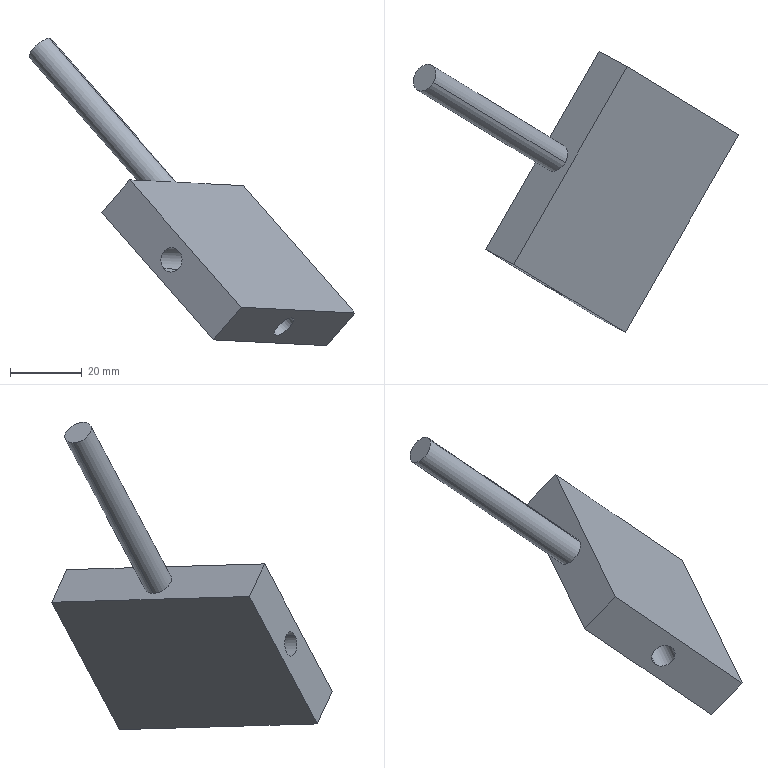Component | SolidWorks | GravitySensorZ0-123-1 | 1 solid | 18 faces | box 90.67 x 78.15 x 85.57 mm | volume 40042 mm3 | cylinder 10 | plane 8 | commonest cylinder face diameters 6.8 x8 8 x2
build123d program:
from build123d import *

# Parameters (mm, degrees)
SKETCH1_W           = 63.5
SKETCH1_H           = 50.8
BOSS_EXTRUDE1_DEPTH = 12.7
M8_TAPPED_HOLE1_D   = 6.8
M8_TAPPED_HOLE2_D   = 6.8
SKETCH6_R           = 4
BOSS_EXTRUDE2_DEPTH = 60


with BuildPart() as part:
    # Sketch1 → Boss-Extrude1 (new body)
    with BuildSketch(Plane.XY):
        Rectangle(SKETCH1_W, SKETCH1_H)
    extrude(amount=BOSS_EXTRUDE1_DEPTH)

    # M8 Tapped Hole1 (through all)
    with Locations(Plane(origin=(31.75, 0, 0), x_dir=(0, 0, -1), z_dir=(1, 0, 0))):
        with Locations((-6.35, 0)):
            Hole(M8_TAPPED_HOLE1_D / 2)

    # M8 Tapped Hole2 (through all)
    with Locations(Plane(origin=(0, 25.4, 0), x_dir=(1, 0, 0), z_dir=(0, 1, 0))):
        with Locations((0, -6.35)):
            Hole(M8_TAPPED_HOLE2_D / 2)

    # Sketch6 → Boss-Extrude2 (add)
    with BuildSketch(Plane.XZ.offset(25.4)):
        with Locations(Location((0, 6.35, 0), (0, 0, 90))):
            Circle(SKETCH6_R)
    extrude(amount=BOSS_EXTRUDE2_DEPTH)


solid = part.part

# Placed as in the assembly
solid = solid.moved(Location((-51.151, -52.012, 80.856), (-155.101, -37.93, -50.876)))
STEP:
#1=COLOUR_RGB('',0.7922,0.8196,0.9333);
#2=FILL_AREA_STYLE_COLOUR('',#1);
#3=FILL_AREA_STYLE('',(#2));
#4=SURFACE_STYLE_FILL_AREA(#3);
#5=SURFACE_SIDE_STYLE('',(#4));
#6=SURFACE_STYLE_USAGE(.BOTH.,#5);
#7=PRESENTATION_STYLE_ASSIGNMENT((#6));
#8=CARTESIAN_POINT('',(-4.128,-0.7677,5.465));
#9=VERTEX_POINT('',#8);
#10=CARTESIAN_POINT('',(-4.322,-0.6631,5.239));
#11=VERTEX_POINT('',#10);
#12=CARTESIAN_POINT('',(-4.225,-0.7154,5.352));
#13=DIRECTION('',(-0.6119,0.3716,0.6982));
#14=DIRECTION('',(0.6147,-0.3321,0.7154));
#15=AXIS2_PLACEMENT_3D('',#12,#13,#14);
#16=CIRCLE('',#15,0.1575);
#17=EDGE_CURVE('',#9,#11,#16,.T.);
#18=ORIENTED_EDGE('',*,*,#17,.F.);
#19=CARTESIAN_POINT('',(-2.683,-1.645,3.815));
#20=VERTEX_POINT('',#19);
#21=CARTESIAN_POINT('',(-4.128,-0.7677,5.465));
#22=DIRECTION('',(0.6119,-0.3716,-0.6982));
#23=VECTOR('',#22,39.37);
#24=LINE('',#21,#23);
#25=EDGE_CURVE('',#9,#20,#24,.T.);
#26=ORIENTED_EDGE('',*,*,#25,.T.);
#27=CARTESIAN_POINT('',(-2.876,-1.541,3.59));
#28=VERTEX_POINT('',#27);
#29=CARTESIAN_POINT('',(-2.779,-1.593,3.703));
#30=DIRECTION('',(-0.6119,0.3716,0.6982));
#31=DIRECTION('',(-0.6147,0.3321,-0.7154));
#32=AXIS2_PLACEMENT_3D('',#29,#30,#31);
#33=CIRCLE('',#32,0.1575);
#34=EDGE_CURVE('',#20,#28,#33,.T.);
#35=ORIENTED_EDGE('',*,*,#34,.T.);
#36=CARTESIAN_POINT('',(-4.322,-0.6631,5.239));
#37=DIRECTION('',(0.6119,-0.3716,-0.6982));
#38=VECTOR('',#37,39.37);
#39=LINE('',#36,#38);
#40=EDGE_CURVE('',#11,#28,#39,.T.);
#41=ORIENTED_EDGE('',*,*,#40,.F.);
#42=EDGE_LOOP('',(#18,#26,#35,#41));
#43=FACE_OUTER_BOUND('',#42,.T.);
#44=CARTESIAN_POINT('',(-4.225,-0.7154,5.352));
#45=DIRECTION('',(0.6119,-0.3716,-0.6982));
#46=DIRECTION('',(-0.6147,0.3321,-0.7154));
#47=AXIS2_PLACEMENT_3D('',#44,#45,#46);
#48=CYLINDRICAL_SURFACE('',#47,0.1575);
#49=ADVANCED_FACE('',(#43),#48,.T.);
#50=CARTESIAN_POINT('',(-2.697,-1.638,3.798));
#51=VERTEX_POINT('',#50);
#52=CARTESIAN_POINT('',(-2.862,-1.549,3.607));
#53=VERTEX_POINT('',#52);
#54=CARTESIAN_POINT('',(-2.779,-1.593,3.703));
#55=DIRECTION('',(0.6119,-0.3716,-0.6982));
#56=DIRECTION('',(-0.6147,0.3321,-0.7154));
#57=AXIS2_PLACEMENT_3D('',#54,#55,#56);
#58=CIRCLE('',#57,0.1339);
#59=EDGE_CURVE('',#51,#53,#58,.T.);
#60=ORIENTED_EDGE('',*,*,#59,.F.);
#61=CARTESIAN_POINT('',(-2.085,-2.009,3.1));
#62=VERTEX_POINT('',#61);
#63=CARTESIAN_POINT('',(-1.473,-2.381,2.402));
#64=DIRECTION('',(0.6119,-0.3716,-0.6982));
#65=VECTOR('',#64,39.37);
#66=LINE('',#63,#65);
#67=EDGE_CURVE('',#51,#62,#66,.T.);
#68=ORIENTED_EDGE('',*,*,#67,.T.);
#69=CARTESIAN_POINT('',(-2.25,-1.92,2.909));
#70=VERTEX_POINT('',#69);
#71=CARTESIAN_POINT('',(-2.25,-1.92,2.909));
#72=CARTESIAN_POINT('',(-2.547,-2.053,3.102));
#73=CARTESIAN_POINT('',(-2.382,-2.142,3.294));
#74=CARTESIAN_POINT('',(-2.085,-2.009,3.1));
#75=(BOUNDED_CURVE()B_SPLINE_CURVE(3,(#71,#72,#73,#74),.UNSPECIFIED.,.F.,.F.)B_SPLINE_CURVE_WITH_KNOTS((4,4),(1.571,4.712),.UNSPECIFIED.)CURVE()GEOMETRIC_REPRESENTATION_ITEM()RATIONAL_B_SPLINE_CURVE((1.,0.3333,0.3333,1.))REPRESENTATION_ITEM(''));
#76=EDGE_CURVE('',#70,#62,#75,.T.);
#77=ORIENTED_EDGE('',*,*,#76,.F.);
#78=CARTESIAN_POINT('',(-1.638,-2.292,2.21));
#79=DIRECTION('',(0.6119,-0.3716,-0.6982));
#80=VECTOR('',#79,39.37);
#81=LINE('',#78,#80);
#82=EDGE_CURVE('',#53,#70,#81,.T.);
#83=ORIENTED_EDGE('',*,*,#82,.F.);
#84=EDGE_LOOP('',(#60,#68,#77,#83));
#85=FACE_OUTER_BOUND('',#84,.T.);
#86=CARTESIAN_POINT('',(-1.556,-2.336,2.306));
#87=DIRECTION('',(0.6119,-0.3716,-0.6982));
#88=DIRECTION('',(-0.6147,0.3321,-0.7154));
#89=AXIS2_PLACEMENT_3D('',#86,#87,#88);
#90=CYLINDRICAL_SURFACE('',#89,0.1339);
#91=ADVANCED_FACE('',(#85),#90,.F.);
#92=CARTESIAN_POINT('',(-2.085,-2.009,3.1));
#93=CARTESIAN_POINT('',(-2.055,-2.341,2.92));
#94=CARTESIAN_POINT('',(-2.219,-2.252,2.729));
#95=CARTESIAN_POINT('',(-2.25,-1.92,2.909));
#96=(BOUNDED_CURVE()B_SPLINE_CURVE(3,(#92,#93,#94,#95),.UNSPECIFIED.,.F.,.F.)B_SPLINE_CURVE_WITH_KNOTS((4,4),(1.571,4.712),.UNSPECIFIED.)CURVE()GEOMETRIC_REPRESENTATION_ITEM()RATIONAL_B_SPLINE_CURVE((1.,0.3333,0.3333,1.))REPRESENTATION_ITEM(''));
#97=EDGE_CURVE('',#62,#70,#96,.T.);
#98=ORIENTED_EDGE('',*,*,#97,.F.);
#99=CARTESIAN_POINT('',(-1.473,-2.381,2.402));
#100=VERTEX_POINT('',#99);
#101=CARTESIAN_POINT('',(-1.473,-2.381,2.402));
#102=DIRECTION('',(0.6119,-0.3716,-0.6982));
#103=VECTOR('',#102,39.37);
#104=LINE('',#101,#103);
#105=EDGE_CURVE('',#62,#100,#104,.T.);
#106=ORIENTED_EDGE('',*,*,#105,.T.);
#107=CARTESIAN_POINT('',(-1.638,-2.292,2.21));
#108=VERTEX_POINT('',#107);
#109=CARTESIAN_POINT('',(-1.556,-2.336,2.306));
#110=DIRECTION('',(0.6119,-0.3716,-0.6982));
#111=DIRECTION('',(-0.6147,0.3321,-0.7154));
#112=AXIS2_PLACEMENT_3D('',#109,#110,#111);
#113=CIRCLE('',#112,0.1339);
#114=EDGE_CURVE('',#100,#108,#113,.T.);
#115=ORIENTED_EDGE('',*,*,#114,.T.);
#116=CARTESIAN_POINT('',(-1.638,-2.292,2.21));
#117=DIRECTION('',(0.6119,-0.3716,-0.6982));
#118=VECTOR('',#117,39.37);
#119=LINE('',#116,#118);
#120=EDGE_CURVE('',#70,#108,#119,.T.);
#121=ORIENTED_EDGE('',*,*,#120,.F.);
#122=EDGE_LOOP('',(#98,#106,#115,#121));
#123=FACE_OUTER_BOUND('',#122,.T.);
#124=CARTESIAN_POINT('',(-1.556,-2.336,2.306));
#125=DIRECTION('',(0.6119,-0.3716,-0.6982));
#126=DIRECTION('',(-0.6147,0.3321,-0.7154));
#127=AXIS2_PLACEMENT_3D('',#124,#125,#126);
#128=CYLINDRICAL_SURFACE('',#127,0.1339);
#129=ADVANCED_FACE('',(#123),#128,.F.);
#130=CARTESIAN_POINT('',(-2.872,-3.004,2.94));
#131=VERTEX_POINT('',#130);
#132=CARTESIAN_POINT('',(-2.707,-3.093,3.132));
#133=VERTEX_POINT('',#132);
#134=CARTESIAN_POINT('',(-2.79,-3.048,3.036));
#135=DIRECTION('',(0.4977,0.867,-0.02519));
#136=DIRECTION('',(0.6147,-0.3321,0.7154));
#137=AXIS2_PLACEMENT_3D('',#134,#135,#136);
#138=CIRCLE('',#137,0.1339);
#139=EDGE_CURVE('',#131,#133,#138,.T.);
#140=ORIENTED_EDGE('',*,*,#139,.F.);
#141=CARTESIAN_POINT('',(-1.628,-0.8365,2.877));
#142=DIRECTION('',(0.4977,0.867,-0.02519));
#143=VECTOR('',#142,39.37);
#144=LINE('',#141,#143);
#145=EDGE_CURVE('',#131,#70,#144,.T.);
#146=ORIENTED_EDGE('',*,*,#145,.T.);
#147=ORIENTED_EDGE('',*,*,#76,.T.);
#148=CARTESIAN_POINT('',(-1.463,-0.9254,3.069));
#149=DIRECTION('',(0.4977,0.867,-0.02519));
#150=VECTOR('',#149,39.37);
#151=LINE('',#148,#150);
#152=EDGE_CURVE('',#133,#62,#151,.T.);
#153=ORIENTED_EDGE('',*,*,#152,.F.);
#154=EDGE_LOOP('',(#140,#146,#147,#153));
#155=FACE_OUTER_BOUND('',#154,.T.);
#156=CARTESIAN_POINT('',(-1.545,-0.881,2.973));
#157=DIRECTION('',(0.4977,0.867,-0.02519));
#158=DIRECTION('',(0.6147,-0.3321,0.7154));
#159=AXIS2_PLACEMENT_3D('',#156,#157,#158);
#160=CYLINDRICAL_SURFACE('',#159,0.1339);
#161=ADVANCED_FACE('',(#155),#160,.F.);
#162=CARTESIAN_POINT('',(-2.085,-2.009,3.1));
#163=CARTESIAN_POINT('',(-2.116,-1.678,3.28));
#164=CARTESIAN_POINT('',(-2.28,-1.589,3.089));
#165=CARTESIAN_POINT('',(-2.25,-1.92,2.909));
#166=(BOUNDED_CURVE()B_SPLINE_CURVE(3,(#162,#163,#164,#165),.UNSPECIFIED.,.F.,.F.)B_SPLINE_CURVE_WITH_KNOTS((4,4),(4.712,7.854),.UNSPECIFIED.)CURVE()GEOMETRIC_REPRESENTATION_ITEM()RATIONAL_B_SPLINE_CURVE((1.,0.3333,0.3333,1.))REPRESENTATION_ITEM(''));
#167=EDGE_CURVE('',#62,#70,#166,.T.);
#168=ORIENTED_EDGE('',*,*,#167,.T.);
#169=CARTESIAN_POINT('',(-1.628,-0.8365,2.877));
#170=VERTEX_POINT('',#169);
#171=CARTESIAN_POINT('',(-1.628,-0.8365,2.877));
#172=DIRECTION('',(0.4977,0.867,-0.02519));
#173=VECTOR('',#172,39.37);
#174=LINE('',#171,#173);
#175=EDGE_CURVE('',#70,#170,#174,.T.);
#176=ORIENTED_EDGE('',*,*,#175,.T.);
#177=CARTESIAN_POINT('',(-1.463,-0.9254,3.069));
#178=VERTEX_POINT('',#177);
#179=CARTESIAN_POINT('',(-1.545,-0.881,2.973));
#180=DIRECTION('',(0.4977,0.867,-0.02519));
#181=DIRECTION('',(0.6147,-0.3321,0.7154));
#182=AXIS2_PLACEMENT_3D('',#179,#180,#181);
#183=CIRCLE('',#182,0.1339);
#184=EDGE_CURVE('',#170,#178,#183,.T.);
#185=ORIENTED_EDGE('',*,*,#184,.T.);
#186=CARTESIAN_POINT('',(-1.463,-0.9254,3.069));
#187=DIRECTION('',(0.4977,0.867,-0.02519));
#188=VECTOR('',#187,39.37);
#189=LINE('',#186,#188);
#190=EDGE_CURVE('',#62,#178,#189,.T.);
#191=ORIENTED_EDGE('',*,*,#190,.F.);
#192=EDGE_LOOP('',(#168,#176,#185,#191));
#193=FACE_OUTER_BOUND('',#192,.T.);
#194=CARTESIAN_POINT('',(-1.545,-0.881,2.973));
#195=DIRECTION('',(0.4977,0.867,-0.02519));
#196=DIRECTION('',(0.6147,-0.3321,0.7154));
#197=AXIS2_PLACEMENT_3D('',#194,#195,#196);
#198=CYLINDRICAL_SURFACE('',#197,0.1339);
#199=ADVANCED_FACE('',(#193),#198,.F.);
#200=CARTESIAN_POINT('',(-3.248,-2.76,3.913));
#201=VERTEX_POINT('',#200);
#202=CARTESIAN_POINT('',(-2.004,-0.5924,3.85));
#203=VERTEX_POINT('',#202);
#204=CARTESIAN_POINT('',(-3.248,-2.76,3.913));
#205=DIRECTION('',(0.4977,0.867,-0.02519));
#206=VECTOR('',#205,39.37);
#207=LINE('',#204,#206);
#208=EDGE_CURVE('',#201,#203,#207,.T.);
#209=ORIENTED_EDGE('',*,*,#208,.T.);
#210=CARTESIAN_POINT('',(-2.311,-0.4264,3.492));
#211=VERTEX_POINT('',#210);
#212=CARTESIAN_POINT('',(-2.311,-0.4264,3.492));
#213=DIRECTION('',(0.6147,-0.3321,0.7154));
#214=VECTOR('',#213,39.37);
#215=LINE('',#212,#214);
#216=EDGE_CURVE('',#211,#203,#215,.T.);
#217=ORIENTED_EDGE('',*,*,#216,.F.);
#218=CARTESIAN_POINT('',(-3.555,-2.594,3.555));
#219=VERTEX_POINT('',#218);
#220=CARTESIAN_POINT('',(-3.555,-2.594,3.555));
#221=DIRECTION('',(0.4977,0.867,-0.02519));
#222=VECTOR('',#221,39.37);
#223=LINE('',#220,#222);
#224=EDGE_CURVE('',#219,#211,#223,.T.);
#225=ORIENTED_EDGE('',*,*,#224,.F.);
#226=CARTESIAN_POINT('',(-3.555,-2.594,3.555));
#227=DIRECTION('',(0.6147,-0.3321,0.7154));
#228=VECTOR('',#227,39.37);
#229=LINE('',#226,#228);
#230=EDGE_CURVE('',#219,#201,#229,.T.);
#231=ORIENTED_EDGE('',*,*,#230,.T.);
#232=EDGE_LOOP('',(#209,#217,#225,#231));
#233=FACE_OUTER_BOUND('',#232,.T.);
#234=CARTESIAN_POINT('',(-2.779,-1.593,3.703));
#235=DIRECTION('',(-0.6119,0.3716,0.6982));
#236=DIRECTION('',(-0.6147,0.3321,-0.7154));
#237=AXIS2_PLACEMENT_3D('',#234,#235,#236);
#238=CIRCLE('',#237,0.1575);
#239=EDGE_CURVE('',#28,#20,#238,.T.);
#240=ORIENTED_EDGE('',*,*,#239,.F.);
#241=ORIENTED_EDGE('',*,*,#34,.F.);
#242=EDGE_LOOP('',(#240,#241));
#243=FACE_BOUND('',#242,.T.);
#244=CARTESIAN_POINT('',(-3.555,-2.594,3.555));
#245=DIRECTION('',(0.6119,-0.3716,-0.6982));
#246=DIRECTION('',(-0.6147,0.3321,-0.7154));
#247=AXIS2_PLACEMENT_3D('',#244,#245,#246);
#248=PLANE('',#247);
#249=ADVANCED_FACE('',(#233,#243),#248,.F.);
#250=ORIENTED_EDGE('',*,*,#175,.F.);
#251=CARTESIAN_POINT('',(-2.25,-1.92,2.909));
#252=CARTESIAN_POINT('',(-1.953,-1.788,2.715));
#253=CARTESIAN_POINT('',(-1.788,-1.877,2.907));
#254=CARTESIAN_POINT('',(-2.085,-2.009,3.1));
#255=(BOUNDED_CURVE()B_SPLINE_CURVE(3,(#251,#252,#253,#254),.UNSPECIFIED.,.F.,.F.)B_SPLINE_CURVE_WITH_KNOTS((4,4),(4.712,7.854),.UNSPECIFIED.)CURVE()GEOMETRIC_REPRESENTATION_ITEM()RATIONAL_B_SPLINE_CURVE((1.,0.3333,0.3333,1.))REPRESENTATION_ITEM(''));
#256=EDGE_CURVE('',#70,#62,#255,.T.);
#257=ORIENTED_EDGE('',*,*,#256,.T.);
#258=ORIENTED_EDGE('',*,*,#190,.T.);
#259=CARTESIAN_POINT('',(-1.545,-0.881,2.973));
#260=DIRECTION('',(0.4977,0.867,-0.02519));
#261=DIRECTION('',(0.6147,-0.3321,0.7154));
#262=AXIS2_PLACEMENT_3D('',#259,#260,#261);
#263=CIRCLE('',#262,0.1339);
#264=EDGE_CURVE('',#178,#170,#263,.T.);
#265=ORIENTED_EDGE('',*,*,#264,.T.);
#266=EDGE_LOOP('',(#250,#257,#258,#265));
#267=FACE_OUTER_BOUND('',#266,.T.);
#268=CARTESIAN_POINT('',(-1.545,-0.881,2.973));
#269=DIRECTION('',(0.4977,0.867,-0.02519));
#270=DIRECTION('',(0.6147,-0.3321,0.7154));
#271=AXIS2_PLACEMENT_3D('',#268,#269,#270);
#272=CYLINDRICAL_SURFACE('',#271,0.1339);
#273=ADVANCED_FACE('',(#267),#272,.F.);
#274=ORIENTED_EDGE('',*,*,#264,.F.);
#275=ORIENTED_EDGE('',*,*,#184,.F.);
#276=EDGE_LOOP('',(#274,#275));
#277=FACE_BOUND('',#276,.T.);
#278=CARTESIAN_POINT('',(-0.7798,-1.336,2.454));
#279=VERTEX_POINT('',#278);
#280=CARTESIAN_POINT('',(-0.7798,-1.336,2.454));
#281=DIRECTION('',(0.6119,-0.3716,-0.6982));
#282=VECTOR('',#281,39.37);
#283=LINE('',#280,#282);
#284=EDGE_CURVE('',#203,#279,#283,.T.);
#285=ORIENTED_EDGE('',*,*,#284,.T.);
#286=CARTESIAN_POINT('',(-1.087,-1.17,2.096));
#287=VERTEX_POINT('',#286);
#288=CARTESIAN_POINT('',(-1.087,-1.17,2.096));
#289=DIRECTION('',(0.6147,-0.3321,0.7154));
#290=VECTOR('',#289,39.37);
#291=LINE('',#288,#290);
#292=EDGE_CURVE('',#287,#279,#291,.T.);
#293=ORIENTED_EDGE('',*,*,#292,.F.);
#294=CARTESIAN_POINT('',(-1.087,-1.17,2.096));
#295=DIRECTION('',(0.6119,-0.3716,-0.6982));
#296=VECTOR('',#295,39.37);
#297=LINE('',#294,#296);
#298=EDGE_CURVE('',#211,#287,#297,.T.);
#299=ORIENTED_EDGE('',*,*,#298,.F.);
#300=ORIENTED_EDGE('',*,*,#216,.T.);
#301=EDGE_LOOP('',(#285,#293,#299,#300));
#302=FACE_OUTER_BOUND('',#301,.T.);
#303=CARTESIAN_POINT('',(-1.087,-1.17,2.096));
#304=DIRECTION('',(-0.4977,-0.867,0.02519));
#305=DIRECTION('',(-0.6119,0.3716,0.6982));
#306=AXIS2_PLACEMENT_3D('',#303,#304,#305);
#307=PLANE('',#306);
#308=ADVANCED_FACE('',(#277,#302),#307,.F.);
#309=CARTESIAN_POINT('',(-1.556,-2.336,2.306));
#310=DIRECTION('',(0.6119,-0.3716,-0.6982));
#311=DIRECTION('',(-0.6147,0.3321,-0.7154));
#312=AXIS2_PLACEMENT_3D('',#309,#310,#311);
#313=CIRCLE('',#312,0.1339);
#314=EDGE_CURVE('',#108,#100,#313,.T.);
#315=ORIENTED_EDGE('',*,*,#314,.F.);
#316=ORIENTED_EDGE('',*,*,#114,.F.);
#317=EDGE_LOOP('',(#315,#316));
#318=FACE_BOUND('',#317,.T.);
#319=CARTESIAN_POINT('',(-2.024,-3.503,2.517));
#320=VERTEX_POINT('',#319);
#321=CARTESIAN_POINT('',(-2.024,-3.503,2.517));
#322=DIRECTION('',(-0.4977,-0.867,0.02519));
#323=VECTOR('',#322,39.37);
#324=LINE('',#321,#323);
#325=EDGE_CURVE('',#279,#320,#324,.T.);
#326=ORIENTED_EDGE('',*,*,#325,.T.);
#327=CARTESIAN_POINT('',(-2.331,-3.337,2.159));
#328=VERTEX_POINT('',#327);
#329=CARTESIAN_POINT('',(-2.331,-3.337,2.159));
#330=DIRECTION('',(0.6147,-0.3321,0.7154));
#331=VECTOR('',#330,39.37);
#332=LINE('',#329,#331);
#333=EDGE_CURVE('',#328,#320,#332,.T.);
#334=ORIENTED_EDGE('',*,*,#333,.F.);
#335=CARTESIAN_POINT('',(-2.331,-3.337,2.159));
#336=DIRECTION('',(-0.4977,-0.867,0.02519));
#337=VECTOR('',#336,39.37);
#338=LINE('',#335,#337);
#339=EDGE_CURVE('',#287,#328,#338,.T.);
#340=ORIENTED_EDGE('',*,*,#339,.F.);
#341=ORIENTED_EDGE('',*,*,#292,.T.);
#342=EDGE_LOOP('',(#326,#334,#340,#341));
#343=FACE_OUTER_BOUND('',#342,.T.);
#344=CARTESIAN_POINT('',(-2.331,-3.337,2.159));
#345=DIRECTION('',(-0.6119,0.3716,0.6982));
#346=DIRECTION('',(0.6147,-0.3321,0.7154));
#347=AXIS2_PLACEMENT_3D('',#344,#345,#346);
#348=PLANE('',#347);
#349=ADVANCED_FACE('',(#318,#343),#348,.F.);
#350=CARTESIAN_POINT('',(-2.79,-3.048,3.036));
#351=DIRECTION('',(0.4977,0.867,-0.02519));
#352=DIRECTION('',(0.6147,-0.3321,0.7154));
#353=AXIS2_PLACEMENT_3D('',#350,#351,#352);
#354=CIRCLE('',#353,0.1339);
#355=EDGE_CURVE('',#133,#131,#354,.T.);
#356=ORIENTED_EDGE('',*,*,#355,.T.);
#357=ORIENTED_EDGE('',*,*,#139,.T.);
#358=EDGE_LOOP('',(#356,#357));
#359=FACE_BOUND('',#358,.T.);
#360=CARTESIAN_POINT('',(-2.024,-3.503,2.517));
#361=DIRECTION('',(-0.6119,0.3716,0.6982));
#362=VECTOR('',#361,39.37);
#363=LINE('',#360,#362);
#364=EDGE_CURVE('',#320,#201,#363,.T.);
#365=ORIENTED_EDGE('',*,*,#364,.T.);
#366=ORIENTED_EDGE('',*,*,#230,.F.);
#367=CARTESIAN_POINT('',(-2.331,-3.337,2.159));
#368=DIRECTION('',(-0.6119,0.3716,0.6982));
#369=VECTOR('',#368,39.37);
#370=LINE('',#367,#369);
#371=EDGE_CURVE('',#328,#219,#370,.T.);
#372=ORIENTED_EDGE('',*,*,#371,.F.);
#373=ORIENTED_EDGE('',*,*,#333,.T.);
#374=EDGE_LOOP('',(#365,#366,#372,#373));
#375=FACE_OUTER_BOUND('',#374,.T.);
#376=CARTESIAN_POINT('',(-2.331,-3.337,2.159));
#377=DIRECTION('',(0.4977,0.867,-0.02519));
#378=DIRECTION('',(0.6119,-0.3716,-0.6982));
#379=AXIS2_PLACEMENT_3D('',#376,#377,#378);
#380=PLANE('',#379);
#381=ADVANCED_FACE('',(#359,#375),#380,.F.);
#382=ORIENTED_EDGE('',*,*,#298,.T.);
#383=ORIENTED_EDGE('',*,*,#339,.T.);
#384=ORIENTED_EDGE('',*,*,#371,.T.);
#385=ORIENTED_EDGE('',*,*,#224,.T.);
#386=EDGE_LOOP('',(#382,#383,#384,#385));
#387=FACE_OUTER_BOUND('',#386,.T.);
#388=CARTESIAN_POINT('',(-2.321,-1.882,2.826));
#389=DIRECTION('',(-0.6147,0.3321,-0.7154));
#390=DIRECTION('',(0.4977,0.867,-0.02519));
#391=AXIS2_PLACEMENT_3D('',#388,#389,#390);
#392=PLANE('',#391);
#393=ADVANCED_FACE('',(#387),#392,.T.);
#394=ORIENTED_EDGE('',*,*,#284,.F.);
#395=ORIENTED_EDGE('',*,*,#208,.F.);
#396=ORIENTED_EDGE('',*,*,#364,.F.);
#397=ORIENTED_EDGE('',*,*,#325,.F.);
#398=EDGE_LOOP('',(#394,#395,#396,#397));
#399=FACE_OUTER_BOUND('',#398,.T.);
#400=CARTESIAN_POINT('',(-2.014,-2.048,3.183));
#401=DIRECTION('',(-0.6147,0.3321,-0.7154));
#402=DIRECTION('',(0.4977,0.867,-0.02519));
#403=AXIS2_PLACEMENT_3D('',#400,#401,#402);
#404=PLANE('',#403);
#405=ADVANCED_FACE('',(#399),#404,.F.);
#406=ORIENTED_EDGE('',*,*,#145,.F.);
#407=ORIENTED_EDGE('',*,*,#355,.F.);
#408=ORIENTED_EDGE('',*,*,#152,.T.);
#409=ORIENTED_EDGE('',*,*,#97,.T.);
#410=EDGE_LOOP('',(#406,#407,#408,#409));
#411=FACE_OUTER_BOUND('',#410,.T.);
#412=CARTESIAN_POINT('',(-1.545,-0.881,2.973));
#413=DIRECTION('',(0.4977,0.867,-0.02519));
#414=DIRECTION('',(0.6147,-0.3321,0.7154));
#415=AXIS2_PLACEMENT_3D('',#412,#413,#414);
#416=CYLINDRICAL_SURFACE('',#415,0.1339);
#417=ADVANCED_FACE('',(#411),#416,.F.);
#418=ORIENTED_EDGE('',*,*,#105,.F.);
#419=ORIENTED_EDGE('',*,*,#256,.F.);
#420=ORIENTED_EDGE('',*,*,#120,.T.);
#421=ORIENTED_EDGE('',*,*,#314,.T.);
#422=EDGE_LOOP('',(#418,#419,#420,#421));
#423=FACE_OUTER_BOUND('',#422,.T.);
#424=CARTESIAN_POINT('',(-1.556,-2.336,2.306));
#425=DIRECTION('',(0.6119,-0.3716,-0.6982));
#426=DIRECTION('',(-0.6147,0.3321,-0.7154));
#427=AXIS2_PLACEMENT_3D('',#424,#425,#426);
#428=CYLINDRICAL_SURFACE('',#427,0.1339);
#429=ADVANCED_FACE('',(#423),#428,.F.);
#430=ORIENTED_EDGE('',*,*,#67,.F.);
#431=CARTESIAN_POINT('',(-2.779,-1.593,3.703));
#432=DIRECTION('',(0.6119,-0.3716,-0.6982));
#433=DIRECTION('',(-0.6147,0.3321,-0.7154));
#434=AXIS2_PLACEMENT_3D('',#431,#432,#433);
#435=CIRCLE('',#434,0.1339);
#436=EDGE_CURVE('',#53,#51,#435,.T.);
#437=ORIENTED_EDGE('',*,*,#436,.F.);
#438=ORIENTED_EDGE('',*,*,#82,.T.);
#439=ORIENTED_EDGE('',*,*,#167,.F.);
#440=EDGE_LOOP('',(#430,#437,#438,#439));
#441=FACE_OUTER_BOUND('',#440,.T.);
#442=CARTESIAN_POINT('',(-1.556,-2.336,2.306));
#443=DIRECTION('',(0.6119,-0.3716,-0.6982));
#444=DIRECTION('',(-0.6147,0.3321,-0.7154));
#445=AXIS2_PLACEMENT_3D('',#442,#443,#444);
#446=CYLINDRICAL_SURFACE('',#445,0.1339);
#447=ADVANCED_FACE('',(#441),#446,.F.);
#448=ORIENTED_EDGE('',*,*,#436,.T.);
#449=ORIENTED_EDGE('',*,*,#59,.T.);
#450=EDGE_LOOP('',(#448,#449));
#451=FACE_OUTER_BOUND('',#450,.T.);
#452=CARTESIAN_POINT('',(-2.779,-1.593,3.703));
#453=DIRECTION('',(-0.6119,0.3716,0.6982));
#454=DIRECTION('',(0.6147,-0.3321,0.7154));
#455=AXIS2_PLACEMENT_3D('',#452,#453,#454);
#456=PLANE('',#455);
#457=ADVANCED_FACE('',(#451),#456,.F.);
#458=ORIENTED_EDGE('',*,*,#25,.F.);
#459=CARTESIAN_POINT('',(-4.225,-0.7154,5.352));
#460=DIRECTION('',(-0.6119,0.3716,0.6982));
#461=DIRECTION('',(0.6147,-0.3321,0.7154));
#462=AXIS2_PLACEMENT_3D('',#459,#460,#461);
#463=CIRCLE('',#462,0.1575);
#464=EDGE_CURVE('',#11,#9,#463,.T.);
#465=ORIENTED_EDGE('',*,*,#464,.F.);
#466=ORIENTED_EDGE('',*,*,#40,.T.);
#467=ORIENTED_EDGE('',*,*,#239,.T.);
#468=EDGE_LOOP('',(#458,#465,#466,#467));
#469=FACE_OUTER_BOUND('',#468,.T.);
#470=CARTESIAN_POINT('',(-4.225,-0.7154,5.352));
#471=DIRECTION('',(0.6119,-0.3716,-0.6982));
#472=DIRECTION('',(-0.6147,0.3321,-0.7154));
#473=AXIS2_PLACEMENT_3D('',#470,#471,#472);
#474=CYLINDRICAL_SURFACE('',#473,0.1575);
#475=ADVANCED_FACE('',(#469),#474,.T.);
#476=ORIENTED_EDGE('',*,*,#464,.T.);
#477=ORIENTED_EDGE('',*,*,#17,.T.);
#478=EDGE_LOOP('',(#476,#477));
#479=FACE_OUTER_BOUND('',#478,.T.);
#480=CARTESIAN_POINT('',(-4.225,-0.7154,5.352));
#481=DIRECTION('',(-0.6119,0.3716,0.6982));
#482=DIRECTION('',(0.6147,-0.3321,0.7154));
#483=AXIS2_PLACEMENT_3D('',#480,#481,#482);
#484=PLANE('',#483);
#485=ADVANCED_FACE('',(#479),#484,.T.);
#486=CLOSED_SHELL('',(#49,#91,#129,#161,#199,#249,#273,#308,#349,#381,#393,#405,#417,#429,#447,#457,#475,#485));
#487=MANIFOLD_SOLID_BREP('',#486);
#488=STYLED_ITEM('',(#7),#487);
#489=PRESENTATION_LAYER_ASSIGNMENT('','',(#488));
#490=(LENGTH_UNIT()NAMED_UNIT(*)SI_UNIT($,.METRE.));
#491=LENGTH_MEASURE_WITH_UNIT(LENGTH_MEASURE(0.0254),#490);
#492=DIMENSIONAL_EXPONENTS(1.,0.,0.,0.,0.,0.,0.);
#493=(CONVERSION_BASED_UNIT('',#491)LENGTH_UNIT()NAMED_UNIT(#492));
#494=UNCERTAINTY_MEASURE_WITH_UNIT(LENGTH_MEASURE(0.00001),#493,'','');
#495=(NAMED_UNIT(*)PLANE_ANGLE_UNIT()SI_UNIT($,.RADIAN.));
#496=(NAMED_UNIT(*)SI_UNIT($,.STERADIAN.)SOLID_ANGLE_UNIT());
#497=(GEOMETRIC_REPRESENTATION_CONTEXT(3)GLOBAL_UNCERTAINTY_ASSIGNED_CONTEXT((#494))GLOBAL_UNIT_ASSIGNED_CONTEXT((#493,#495,#496))REPRESENTATION_CONTEXT('',''));
#498=MECHANICAL_DESIGN_GEOMETRIC_PRESENTATION_REPRESENTATION('',(#488),#497);
#499=CARTESIAN_POINT('',(0.,0.,0.));
#500=DIRECTION('',(0.,0.,1.));
#501=DIRECTION('',(1.,0.,0.));
#502=AXIS2_PLACEMENT_3D('',#499,#500,#501);
#503=(LENGTH_UNIT()NAMED_UNIT(*)SI_UNIT($,.METRE.));
#504=LENGTH_MEASURE_WITH_UNIT(LENGTH_MEASURE(0.0254),#503);
#505=DIMENSIONAL_EXPONENTS(1.,0.,0.,0.,0.,0.,0.);
#506=(CONVERSION_BASED_UNIT('',#504)LENGTH_UNIT()NAMED_UNIT(#505));
#507=UNCERTAINTY_MEASURE_WITH_UNIT(LENGTH_MEASURE(0.00001),#506,'','');
#508=(NAMED_UNIT(*)PLANE_ANGLE_UNIT()SI_UNIT($,.RADIAN.));
#509=(NAMED_UNIT(*)SI_UNIT($,.STERADIAN.)SOLID_ANGLE_UNIT());
#510=(GEOMETRIC_REPRESENTATION_CONTEXT(3)GLOBAL_UNCERTAINTY_ASSIGNED_CONTEXT((#507))GLOBAL_UNIT_ASSIGNED_CONTEXT((#506,#508,#509))REPRESENTATION_CONTEXT('',''));
#511=ADVANCED_BREP_SHAPE_REPRESENTATION('',(#487,#502),#510);